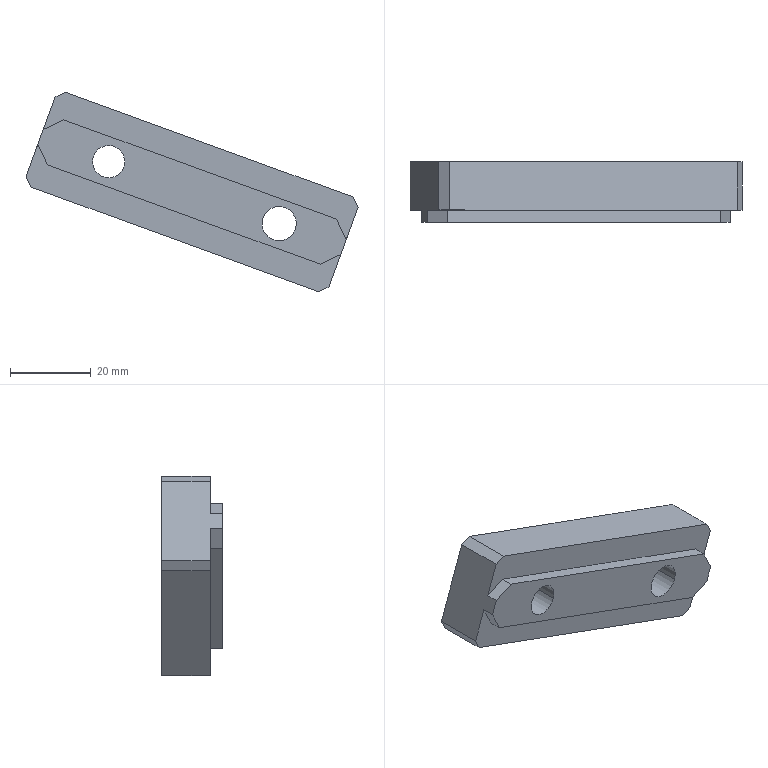Component | SolidWorks | MA060.03.03-06-8 | 1 solid | 22 faces | box 82.36 x 15 x 49.49 mm | volume 25059 mm3 | plane 18 | cylinder 4 | commonest cylinder face diameters 8.5 x2 8 x2 | material Q235A
STEP:
#1=COLOUR_RGB('',0.7922,0.8196,0.9333);
#2=FILL_AREA_STYLE_COLOUR('',#1);
#3=FILL_AREA_STYLE('',(#2));
#4=SURFACE_STYLE_FILL_AREA(#3);
#5=SURFACE_SIDE_STYLE('',(#4));
#6=SURFACE_STYLE_USAGE(.BOTH.,#5);
#7=PRESENTATION_STYLE_ASSIGNMENT((#6));
#8=CARTESIAN_POINT('',(-8.875,3.427,3.232));
#9=VERTEX_POINT('',#8);
#10=CARTESIAN_POINT('',(-8.56,3.427,3.118));
#11=VERTEX_POINT('',#10);
#12=CARTESIAN_POINT('',(-8.718,3.427,3.175));
#13=DIRECTION('',(-0.,1.,0.));
#14=DIRECTION('',(0.9397,0.,-0.342));
#15=AXIS2_PLACEMENT_3D('',#12,#13,#14);
#16=CIRCLE('',#15,0.1673);
#17=EDGE_CURVE('',#9,#11,#16,.T.);
#18=ORIENTED_EDGE('',*,*,#17,.F.);
#19=CARTESIAN_POINT('',(-8.875,4.018,3.232));
#20=VERTEX_POINT('',#19);
#21=CARTESIAN_POINT('',(-8.875,3.427,3.232));
#22=DIRECTION('',(-0.,1.,0.));
#23=VECTOR('',#22,39.37);
#24=LINE('',#21,#23);
#25=EDGE_CURVE('',#9,#20,#24,.T.);
#26=ORIENTED_EDGE('',*,*,#25,.T.);
#27=CARTESIAN_POINT('',(-8.56,4.018,3.118));
#28=VERTEX_POINT('',#27);
#29=CARTESIAN_POINT('',(-8.718,4.018,3.175));
#30=DIRECTION('',(-0.,1.,0.));
#31=DIRECTION('',(0.9397,0.,-0.342));
#32=AXIS2_PLACEMENT_3D('',#29,#30,#31);
#33=CIRCLE('',#32,0.1673);
#34=EDGE_CURVE('',#20,#28,#33,.T.);
#35=ORIENTED_EDGE('',*,*,#34,.T.);
#36=CARTESIAN_POINT('',(-8.56,3.427,3.118));
#37=DIRECTION('',(-0.,1.,0.));
#38=VECTOR('',#37,39.37);
#39=LINE('',#36,#38);
#40=EDGE_CURVE('',#11,#28,#39,.T.);
#41=ORIENTED_EDGE('',*,*,#40,.F.);
#42=EDGE_LOOP('',(#18,#26,#35,#41));
#43=FACE_OUTER_BOUND('',#42,.T.);
#44=CARTESIAN_POINT('',(-8.718,3.427,3.175));
#45=DIRECTION('',(-0.,1.,0.));
#46=DIRECTION('',(0.9397,0.,-0.342));
#47=AXIS2_PLACEMENT_3D('',#44,#45,#46);
#48=CYLINDRICAL_SURFACE('',#47,0.1673);
#49=ADVANCED_FACE('',(#43),#48,.F.);
#50=CARTESIAN_POINT('',(-10.53,3.427,3.835));
#51=VERTEX_POINT('',#50);
#52=CARTESIAN_POINT('',(-10.234,3.427,3.727));
#53=VERTEX_POINT('',#52);
#54=CARTESIAN_POINT('',(-10.382,3.427,3.781));
#55=DIRECTION('',(-0.,1.,0.));
#56=DIRECTION('',(0.9397,0.,-0.342));
#57=AXIS2_PLACEMENT_3D('',#54,#55,#56);
#58=CIRCLE('',#57,0.1575);
#59=EDGE_CURVE('',#51,#53,#58,.T.);
#60=ORIENTED_EDGE('',*,*,#59,.F.);
#61=CARTESIAN_POINT('',(-10.53,4.018,3.835));
#62=VERTEX_POINT('',#61);
#63=CARTESIAN_POINT('',(-10.53,4.018,3.835));
#64=DIRECTION('',(-0.,1.,0.));
#65=VECTOR('',#64,39.37);
#66=LINE('',#63,#65);
#67=EDGE_CURVE('',#51,#62,#66,.T.);
#68=ORIENTED_EDGE('',*,*,#67,.T.);
#69=CARTESIAN_POINT('',(-10.234,4.018,3.727));
#70=VERTEX_POINT('',#69);
#71=CARTESIAN_POINT('',(-10.382,4.018,3.781));
#72=DIRECTION('',(-0.,1.,0.));
#73=DIRECTION('',(0.9397,0.,-0.342));
#74=AXIS2_PLACEMENT_3D('',#71,#72,#73);
#75=CIRCLE('',#74,0.1575);
#76=EDGE_CURVE('',#62,#70,#75,.T.);
#77=ORIENTED_EDGE('',*,*,#76,.T.);
#78=CARTESIAN_POINT('',(-10.234,4.018,3.727));
#79=DIRECTION('',(-0.,1.,0.));
#80=VECTOR('',#79,39.37);
#81=LINE('',#78,#80);
#82=EDGE_CURVE('',#53,#70,#81,.T.);
#83=ORIENTED_EDGE('',*,*,#82,.F.);
#84=EDGE_LOOP('',(#60,#68,#77,#83));
#85=FACE_OUTER_BOUND('',#84,.T.);
#86=CARTESIAN_POINT('',(-10.382,4.018,3.781));
#87=DIRECTION('',(-0.,1.,0.));
#88=DIRECTION('',(0.9397,0.,-0.342));
#89=AXIS2_PLACEMENT_3D('',#86,#87,#88);
#90=CYLINDRICAL_SURFACE('',#89,0.1575);
#91=ADVANCED_FACE('',(#85),#90,.F.);
#92=CARTESIAN_POINT('',(-8.718,3.427,3.175));
#93=DIRECTION('',(-0.,1.,0.));
#94=DIRECTION('',(0.9397,0.,-0.342));
#95=AXIS2_PLACEMENT_3D('',#92,#93,#94);
#96=CIRCLE('',#95,0.1673);
#97=EDGE_CURVE('',#11,#9,#96,.T.);
#98=ORIENTED_EDGE('',*,*,#97,.T.);
#99=ORIENTED_EDGE('',*,*,#17,.T.);
#100=EDGE_LOOP('',(#98,#99));
#101=FACE_BOUND('',#100,.T.);
#102=CARTESIAN_POINT('',(-10.382,3.427,3.781));
#103=DIRECTION('',(-0.,1.,0.));
#104=DIRECTION('',(0.9397,0.,-0.342));
#105=AXIS2_PLACEMENT_3D('',#102,#103,#104);
#106=CIRCLE('',#105,0.1575);
#107=EDGE_CURVE('',#53,#51,#106,.T.);
#108=ORIENTED_EDGE('',*,*,#107,.T.);
#109=ORIENTED_EDGE('',*,*,#59,.T.);
#110=EDGE_LOOP('',(#108,#109));
#111=FACE_BOUND('',#110,.T.);
#112=CARTESIAN_POINT('',(-11.075,3.427,3.951));
#113=VERTEX_POINT('',#112);
#114=CARTESIAN_POINT('',(-11.022,3.427,4.095));
#115=VERTEX_POINT('',#114);
#116=CARTESIAN_POINT('',(-10.88,3.427,4.486));
#117=DIRECTION('',(0.342,0.,0.9397));
#118=VECTOR('',#117,39.37);
#119=LINE('',#116,#118);
#120=EDGE_CURVE('',#113,#115,#119,.T.);
#121=ORIENTED_EDGE('',*,*,#120,.F.);
#122=CARTESIAN_POINT('',(-10.98,3.427,3.749));
#123=VERTEX_POINT('',#122);
#124=CARTESIAN_POINT('',(-11.086,3.427,3.976));
#125=DIRECTION('',(0.4226,0.,-0.9063));
#126=VECTOR('',#125,39.37);
#127=LINE('',#124,#126);
#128=EDGE_CURVE('',#113,#123,#127,.T.);
#129=ORIENTED_EDGE('',*,*,#128,.T.);
#130=CARTESIAN_POINT('',(-8.317,3.427,2.78));
#131=VERTEX_POINT('',#130);
#132=CARTESIAN_POINT('',(-11.128,3.427,3.803));
#133=DIRECTION('',(0.9397,0.,-0.342));
#134=VECTOR('',#133,39.37);
#135=LINE('',#132,#134);
#136=EDGE_CURVE('',#123,#131,#135,.T.);
#137=ORIENTED_EDGE('',*,*,#136,.T.);
#138=CARTESIAN_POINT('',(-8.115,3.427,2.874));
#139=VERTEX_POINT('',#138);
#140=CARTESIAN_POINT('',(-8.09,3.427,2.886));
#141=DIRECTION('',(0.9063,0.,0.4226));
#142=VECTOR('',#141,39.37);
#143=LINE('',#140,#142);
#144=EDGE_CURVE('',#131,#139,#143,.T.);
#145=ORIENTED_EDGE('',*,*,#144,.T.);
#146=CARTESIAN_POINT('',(-8.062,3.427,3.018));
#147=VERTEX_POINT('',#146);
#148=CARTESIAN_POINT('',(-7.92,3.427,3.409));
#149=DIRECTION('',(-0.342,-0.,-0.9397));
#150=VECTOR('',#149,39.37);
#151=LINE('',#148,#150);
#152=EDGE_CURVE('',#147,#139,#151,.T.);
#153=ORIENTED_EDGE('',*,*,#152,.F.);
#154=CARTESIAN_POINT('',(-8.156,3.427,3.22));
#155=VERTEX_POINT('',#154);
#156=CARTESIAN_POINT('',(-8.051,3.427,2.993));
#157=DIRECTION('',(-0.4226,-0.,0.9063));
#158=VECTOR('',#157,39.37);
#159=LINE('',#156,#158);
#160=EDGE_CURVE('',#147,#155,#159,.T.);
#161=ORIENTED_EDGE('',*,*,#160,.T.);
#162=CARTESIAN_POINT('',(-10.82,3.427,4.19));
#163=VERTEX_POINT('',#162);
#164=CARTESIAN_POINT('',(-10.968,3.427,4.243));
#165=DIRECTION('',(0.9397,0.,-0.342));
#166=VECTOR('',#165,39.37);
#167=LINE('',#164,#166);
#168=EDGE_CURVE('',#163,#155,#167,.T.);
#169=ORIENTED_EDGE('',*,*,#168,.F.);
#170=CARTESIAN_POINT('',(-11.047,3.427,4.084));
#171=DIRECTION('',(-0.9063,-0.,-0.4226));
#172=VECTOR('',#171,39.37);
#173=LINE('',#170,#172);
#174=EDGE_CURVE('',#163,#115,#173,.T.);
#175=ORIENTED_EDGE('',*,*,#174,.T.);
#176=EDGE_LOOP('',(#121,#129,#137,#145,#153,#161,#169,#175));
#177=FACE_OUTER_BOUND('',#176,.T.);
#178=CARTESIAN_POINT('',(-9.568,3.427,3.485));
#179=DIRECTION('',(0.,-1.,-0.));
#180=DIRECTION('',(-0.9397,-0.,0.342));
#181=AXIS2_PLACEMENT_3D('',#178,#179,#180);
#182=PLANE('',#181);
#183=ADVANCED_FACE('',(#101,#111,#177),#182,.T.);
#184=CARTESIAN_POINT('',(-8.062,3.545,3.018));
#185=VERTEX_POINT('',#184);
#186=CARTESIAN_POINT('',(-8.062,4.018,3.018));
#187=DIRECTION('',(-0.,1.,0.));
#188=VECTOR('',#187,39.37);
#189=LINE('',#186,#188);
#190=EDGE_CURVE('',#147,#185,#189,.T.);
#191=ORIENTED_EDGE('',*,*,#190,.F.);
#192=ORIENTED_EDGE('',*,*,#152,.T.);
#193=CARTESIAN_POINT('',(-8.115,3.545,2.874));
#194=VERTEX_POINT('',#193);
#195=CARTESIAN_POINT('',(-8.115,4.018,2.874));
#196=DIRECTION('',(0.,-1.,-0.));
#197=VECTOR('',#196,39.37);
#198=LINE('',#195,#197);
#199=EDGE_CURVE('',#194,#139,#198,.T.);
#200=ORIENTED_EDGE('',*,*,#199,.F.);
#201=CARTESIAN_POINT('',(-8.23,3.545,2.558));
#202=VERTEX_POINT('',#201);
#203=CARTESIAN_POINT('',(-8.257,3.545,2.484));
#204=DIRECTION('',(0.342,-0.,0.9397));
#205=VECTOR('',#204,39.37);
#206=LINE('',#203,#205);
#207=EDGE_CURVE('',#202,#194,#206,.T.);
#208=ORIENTED_EDGE('',*,*,#207,.F.);
#209=CARTESIAN_POINT('',(-8.23,4.018,2.558));
#210=VERTEX_POINT('',#209);
#211=CARTESIAN_POINT('',(-8.23,4.018,2.558));
#212=DIRECTION('',(-0.,1.,0.));
#213=VECTOR('',#212,39.37);
#214=LINE('',#211,#213);
#215=EDGE_CURVE('',#202,#210,#214,.T.);
#216=ORIENTED_EDGE('',*,*,#215,.T.);
#217=CARTESIAN_POINT('',(-7.947,4.018,3.335));
#218=VERTEX_POINT('',#217);
#219=CARTESIAN_POINT('',(-7.92,4.018,3.409));
#220=DIRECTION('',(-0.342,-0.,-0.9397));
#221=VECTOR('',#220,39.37);
#222=LINE('',#219,#221);
#223=EDGE_CURVE('',#218,#210,#222,.T.);
#224=ORIENTED_EDGE('',*,*,#223,.F.);
#225=CARTESIAN_POINT('',(-7.947,3.545,3.335));
#226=VERTEX_POINT('',#225);
#227=CARTESIAN_POINT('',(-7.947,4.018,3.335));
#228=DIRECTION('',(0.,-1.,-0.));
#229=VECTOR('',#228,39.37);
#230=LINE('',#227,#229);
#231=EDGE_CURVE('',#218,#226,#230,.T.);
#232=ORIENTED_EDGE('',*,*,#231,.T.);
#233=CARTESIAN_POINT('',(-7.92,3.545,3.409));
#234=DIRECTION('',(0.342,0.,0.9397));
#235=VECTOR('',#234,39.37);
#236=LINE('',#233,#235);
#237=EDGE_CURVE('',#185,#226,#236,.T.);
#238=ORIENTED_EDGE('',*,*,#237,.F.);
#239=EDGE_LOOP('',(#191,#192,#200,#208,#216,#224,#232,#238));
#240=FACE_OUTER_BOUND('',#239,.T.);
#241=CARTESIAN_POINT('',(-7.92,4.018,3.409));
#242=DIRECTION('',(-0.9397,-0.,0.342));
#243=DIRECTION('',(-0.,1.,0.));
#244=AXIS2_PLACEMENT_3D('',#241,#242,#243);
#245=PLANE('',#244);
#246=ADVANCED_FACE('',(#240),#245,.F.);
#247=CARTESIAN_POINT('',(-11.075,3.545,3.951));
#248=VERTEX_POINT('',#247);
#249=CARTESIAN_POINT('',(-11.075,4.018,3.951));
#250=DIRECTION('',(-0.,1.,0.));
#251=VECTOR('',#250,39.37);
#252=LINE('',#249,#251);
#253=EDGE_CURVE('',#113,#248,#252,.T.);
#254=ORIENTED_EDGE('',*,*,#253,.F.);
#255=ORIENTED_EDGE('',*,*,#120,.T.);
#256=CARTESIAN_POINT('',(-11.022,3.545,4.095));
#257=VERTEX_POINT('',#256);
#258=CARTESIAN_POINT('',(-11.022,4.018,4.095));
#259=DIRECTION('',(0.,-1.,-0.));
#260=VECTOR('',#259,39.37);
#261=LINE('',#258,#260);
#262=EDGE_CURVE('',#257,#115,#261,.T.);
#263=ORIENTED_EDGE('',*,*,#262,.F.);
#264=CARTESIAN_POINT('',(-10.907,3.545,4.412));
#265=VERTEX_POINT('',#264);
#266=CARTESIAN_POINT('',(-10.88,3.545,4.486));
#267=DIRECTION('',(0.342,0.,0.9397));
#268=VECTOR('',#267,39.37);
#269=LINE('',#266,#268);
#270=EDGE_CURVE('',#257,#265,#269,.T.);
#271=ORIENTED_EDGE('',*,*,#270,.T.);
#272=CARTESIAN_POINT('',(-10.907,4.018,4.412));
#273=VERTEX_POINT('',#272);
#274=CARTESIAN_POINT('',(-10.907,4.018,4.412));
#275=DIRECTION('',(-0.,1.,0.));
#276=VECTOR('',#275,39.37);
#277=LINE('',#274,#276);
#278=EDGE_CURVE('',#265,#273,#277,.T.);
#279=ORIENTED_EDGE('',*,*,#278,.T.);
#280=CARTESIAN_POINT('',(-11.19,4.018,3.635));
#281=VERTEX_POINT('',#280);
#282=CARTESIAN_POINT('',(-10.88,4.018,4.486));
#283=DIRECTION('',(0.342,0.,0.9397));
#284=VECTOR('',#283,39.37);
#285=LINE('',#282,#284);
#286=EDGE_CURVE('',#281,#273,#285,.T.);
#287=ORIENTED_EDGE('',*,*,#286,.F.);
#288=CARTESIAN_POINT('',(-11.19,3.545,3.635));
#289=VERTEX_POINT('',#288);
#290=CARTESIAN_POINT('',(-11.19,4.018,3.635));
#291=DIRECTION('',(0.,-1.,-0.));
#292=VECTOR('',#291,39.37);
#293=LINE('',#290,#292);
#294=EDGE_CURVE('',#281,#289,#293,.T.);
#295=ORIENTED_EDGE('',*,*,#294,.T.);
#296=CARTESIAN_POINT('',(-11.217,3.545,3.561));
#297=DIRECTION('',(0.342,-0.,0.9397));
#298=VECTOR('',#297,39.37);
#299=LINE('',#296,#298);
#300=EDGE_CURVE('',#289,#248,#299,.T.);
#301=ORIENTED_EDGE('',*,*,#300,.T.);
#302=EDGE_LOOP('',(#254,#255,#263,#271,#279,#287,#295,#301));
#303=FACE_OUTER_BOUND('',#302,.T.);
#304=CARTESIAN_POINT('',(-10.88,4.018,4.486));
#305=DIRECTION('',(0.9397,0.,-0.342));
#306=DIRECTION('',(0.,-1.,-0.));
#307=AXIS2_PLACEMENT_3D('',#304,#305,#306);
#308=PLANE('',#307);
#309=ADVANCED_FACE('',(#303),#308,.F.);
#310=CARTESIAN_POINT('',(-10.98,3.545,3.749));
#311=VERTEX_POINT('',#310);
#312=CARTESIAN_POINT('',(-10.98,3.427,3.749));
#313=DIRECTION('',(0.,-1.,-0.));
#314=VECTOR('',#313,39.37);
#315=LINE('',#312,#314);
#316=EDGE_CURVE('',#311,#123,#315,.T.);
#317=ORIENTED_EDGE('',*,*,#316,.F.);
#318=CARTESIAN_POINT('',(-8.317,3.545,2.78));
#319=VERTEX_POINT('',#318);
#320=CARTESIAN_POINT('',(-11.128,3.545,3.803));
#321=DIRECTION('',(0.9397,0.,-0.342));
#322=VECTOR('',#321,39.37);
#323=LINE('',#320,#322);
#324=EDGE_CURVE('',#311,#319,#323,.T.);
#325=ORIENTED_EDGE('',*,*,#324,.T.);
#326=CARTESIAN_POINT('',(-8.317,3.427,2.78));
#327=DIRECTION('',(-0.,1.,0.));
#328=VECTOR('',#327,39.37);
#329=LINE('',#326,#328);
#330=EDGE_CURVE('',#131,#319,#329,.T.);
#331=ORIENTED_EDGE('',*,*,#330,.F.);
#332=ORIENTED_EDGE('',*,*,#136,.F.);
#333=EDGE_LOOP('',(#317,#325,#331,#332));
#334=FACE_OUTER_BOUND('',#333,.T.);
#335=CARTESIAN_POINT('',(-11.128,3.427,3.803));
#336=DIRECTION('',(0.342,0.,0.9397));
#337=DIRECTION('',(0.,-1.,-0.));
#338=AXIS2_PLACEMENT_3D('',#335,#336,#337);
#339=PLANE('',#338);
#340=ADVANCED_FACE('',(#334),#339,.F.);
#341=CARTESIAN_POINT('',(-8.156,3.545,3.22));
#342=VERTEX_POINT('',#341);
#343=CARTESIAN_POINT('',(-8.156,3.427,3.22));
#344=DIRECTION('',(0.,-1.,-0.));
#345=VECTOR('',#344,39.37);
#346=LINE('',#343,#345);
#347=EDGE_CURVE('',#342,#155,#346,.T.);
#348=ORIENTED_EDGE('',*,*,#347,.F.);
#349=CARTESIAN_POINT('',(-10.82,3.545,4.19));
#350=VERTEX_POINT('',#349);
#351=CARTESIAN_POINT('',(-10.968,3.545,4.243));
#352=DIRECTION('',(0.9397,0.,-0.342));
#353=VECTOR('',#352,39.37);
#354=LINE('',#351,#353);
#355=EDGE_CURVE('',#350,#342,#354,.T.);
#356=ORIENTED_EDGE('',*,*,#355,.F.);
#357=CARTESIAN_POINT('',(-10.82,3.427,4.19));
#358=DIRECTION('',(-0.,1.,0.));
#359=VECTOR('',#358,39.37);
#360=LINE('',#357,#359);
#361=EDGE_CURVE('',#163,#350,#360,.T.);
#362=ORIENTED_EDGE('',*,*,#361,.F.);
#363=ORIENTED_EDGE('',*,*,#168,.T.);
#364=EDGE_LOOP('',(#348,#356,#362,#363));
#365=FACE_OUTER_BOUND('',#364,.T.);
#366=CARTESIAN_POINT('',(-10.968,3.427,4.243));
#367=DIRECTION('',(-0.342,-0.,-0.9397));
#368=DIRECTION('',(-0.,1.,0.));
#369=AXIS2_PLACEMENT_3D('',#366,#367,#368);
#370=PLANE('',#369);
#371=ADVANCED_FACE('',(#365),#370,.F.);
#372=CARTESIAN_POINT('',(-11.143,3.545,3.534));
#373=VERTEX_POINT('',#372);
#374=CARTESIAN_POINT('',(-8.331,3.545,2.511));
#375=VERTEX_POINT('',#374);
#376=CARTESIAN_POINT('',(-11.217,3.545,3.561));
#377=DIRECTION('',(0.9397,0.,-0.342));
#378=VECTOR('',#377,39.37);
#379=LINE('',#376,#378);
#380=EDGE_CURVE('',#373,#375,#379,.T.);
#381=ORIENTED_EDGE('',*,*,#380,.F.);
#382=CARTESIAN_POINT('',(-11.143,4.018,3.534));
#383=VERTEX_POINT('',#382);
#384=CARTESIAN_POINT('',(-11.143,4.018,3.534));
#385=DIRECTION('',(-0.,1.,0.));
#386=VECTOR('',#385,39.37);
#387=LINE('',#384,#386);
#388=EDGE_CURVE('',#373,#383,#387,.T.);
#389=ORIENTED_EDGE('',*,*,#388,.T.);
#390=CARTESIAN_POINT('',(-8.331,4.018,2.511));
#391=VERTEX_POINT('',#390);
#392=CARTESIAN_POINT('',(-11.217,4.018,3.561));
#393=DIRECTION('',(-0.9397,-0.,0.342));
#394=VECTOR('',#393,39.37);
#395=LINE('',#392,#394);
#396=EDGE_CURVE('',#391,#383,#395,.T.);
#397=ORIENTED_EDGE('',*,*,#396,.F.);
#398=CARTESIAN_POINT('',(-8.331,4.018,2.511));
#399=DIRECTION('',(0.,-1.,-0.));
#400=VECTOR('',#399,39.37);
#401=LINE('',#398,#400);
#402=EDGE_CURVE('',#391,#375,#401,.T.);
#403=ORIENTED_EDGE('',*,*,#402,.T.);
#404=EDGE_LOOP('',(#381,#389,#397,#403));
#405=FACE_OUTER_BOUND('',#404,.T.);
#406=CARTESIAN_POINT('',(-11.217,4.018,3.561));
#407=DIRECTION('',(0.342,0.,0.9397));
#408=DIRECTION('',(0.,-1.,-0.));
#409=AXIS2_PLACEMENT_3D('',#406,#407,#408);
#410=PLANE('',#409);
#411=ADVANCED_FACE('',(#405),#410,.F.);
#412=CARTESIAN_POINT('',(-10.806,4.018,4.459));
#413=VERTEX_POINT('',#412);
#414=CARTESIAN_POINT('',(-7.994,4.018,3.435));
#415=VERTEX_POINT('',#414);
#416=CARTESIAN_POINT('',(-10.88,4.018,4.486));
#417=DIRECTION('',(0.9397,0.,-0.342));
#418=VECTOR('',#417,39.37);
#419=LINE('',#416,#418);
#420=EDGE_CURVE('',#413,#415,#419,.T.);
#421=ORIENTED_EDGE('',*,*,#420,.F.);
#422=CARTESIAN_POINT('',(-10.806,3.545,4.459));
#423=VERTEX_POINT('',#422);
#424=CARTESIAN_POINT('',(-10.806,4.018,4.459));
#425=DIRECTION('',(0.,-1.,-0.));
#426=VECTOR('',#425,39.37);
#427=LINE('',#424,#426);
#428=EDGE_CURVE('',#413,#423,#427,.T.);
#429=ORIENTED_EDGE('',*,*,#428,.T.);
#430=CARTESIAN_POINT('',(-7.994,3.545,3.435));
#431=VERTEX_POINT('',#430);
#432=CARTESIAN_POINT('',(-10.88,3.545,4.486));
#433=DIRECTION('',(0.9397,0.,-0.342));
#434=VECTOR('',#433,39.37);
#435=LINE('',#432,#434);
#436=EDGE_CURVE('',#423,#431,#435,.T.);
#437=ORIENTED_EDGE('',*,*,#436,.T.);
#438=CARTESIAN_POINT('',(-7.994,4.018,3.435));
#439=DIRECTION('',(-0.,1.,0.));
#440=VECTOR('',#439,39.37);
#441=LINE('',#438,#440);
#442=EDGE_CURVE('',#431,#415,#441,.T.);
#443=ORIENTED_EDGE('',*,*,#442,.T.);
#444=EDGE_LOOP('',(#421,#429,#437,#443));
#445=FACE_OUTER_BOUND('',#444,.T.);
#446=CARTESIAN_POINT('',(-10.88,4.018,4.486));
#447=DIRECTION('',(-0.342,-0.,-0.9397));
#448=DIRECTION('',(-0.,1.,0.));
#449=AXIS2_PLACEMENT_3D('',#446,#447,#448);
#450=PLANE('',#449);
#451=ADVANCED_FACE('',(#445),#450,.F.);
#452=CARTESIAN_POINT('',(-8.718,4.018,3.175));
#453=DIRECTION('',(-0.,1.,0.));
#454=DIRECTION('',(0.9397,0.,-0.342));
#455=AXIS2_PLACEMENT_3D('',#452,#453,#454);
#456=CIRCLE('',#455,0.1673);
#457=EDGE_CURVE('',#28,#20,#456,.T.);
#458=ORIENTED_EDGE('',*,*,#457,.F.);
#459=ORIENTED_EDGE('',*,*,#34,.F.);
#460=EDGE_LOOP('',(#458,#459));
#461=FACE_BOUND('',#460,.T.);
#462=CARTESIAN_POINT('',(-10.382,4.018,3.781));
#463=DIRECTION('',(-0.,1.,0.));
#464=DIRECTION('',(0.9397,0.,-0.342));
#465=AXIS2_PLACEMENT_3D('',#462,#463,#464);
#466=CIRCLE('',#465,0.1575);
#467=EDGE_CURVE('',#70,#62,#466,.T.);
#468=ORIENTED_EDGE('',*,*,#467,.F.);
#469=ORIENTED_EDGE('',*,*,#76,.F.);
#470=EDGE_LOOP('',(#468,#469));
#471=FACE_BOUND('',#470,.T.);
#472=ORIENTED_EDGE('',*,*,#286,.T.);
#473=CARTESIAN_POINT('',(-10.806,4.018,4.459));
#474=DIRECTION('',(0.9063,0.,0.4226));
#475=VECTOR('',#474,39.37);
#476=LINE('',#473,#475);
#477=EDGE_CURVE('',#273,#413,#476,.T.);
#478=ORIENTED_EDGE('',*,*,#477,.T.);
#479=ORIENTED_EDGE('',*,*,#420,.T.);
#480=CARTESIAN_POINT('',(-7.947,4.018,3.335));
#481=DIRECTION('',(0.4226,0.,-0.9063));
#482=VECTOR('',#481,39.37);
#483=LINE('',#480,#482);
#484=EDGE_CURVE('',#415,#218,#483,.T.);
#485=ORIENTED_EDGE('',*,*,#484,.T.);
#486=ORIENTED_EDGE('',*,*,#223,.T.);
#487=CARTESIAN_POINT('',(-8.331,4.018,2.511));
#488=DIRECTION('',(-0.9063,-0.,-0.4226));
#489=VECTOR('',#488,39.37);
#490=LINE('',#487,#489);
#491=EDGE_CURVE('',#210,#391,#490,.T.);
#492=ORIENTED_EDGE('',*,*,#491,.T.);
#493=ORIENTED_EDGE('',*,*,#396,.T.);
#494=CARTESIAN_POINT('',(-11.19,4.018,3.635));
#495=DIRECTION('',(-0.4226,-0.,0.9063));
#496=VECTOR('',#495,39.37);
#497=LINE('',#494,#496);
#498=EDGE_CURVE('',#383,#281,#497,.T.);
#499=ORIENTED_EDGE('',*,*,#498,.T.);
#500=EDGE_LOOP('',(#472,#478,#479,#485,#486,#492,#493,#499));
#501=FACE_OUTER_BOUND('',#500,.T.);
#502=CARTESIAN_POINT('',(-9.568,4.018,3.485));
#503=DIRECTION('',(0.,-1.,-0.));
#504=DIRECTION('',(-0.9397,-0.,0.342));
#505=AXIS2_PLACEMENT_3D('',#502,#503,#504);
#506=PLANE('',#505);
#507=ADVANCED_FACE('',(#461,#471,#501),#506,.F.);
#508=ORIENTED_EDGE('',*,*,#67,.F.);
#509=ORIENTED_EDGE('',*,*,#107,.F.);
#510=ORIENTED_EDGE('',*,*,#82,.T.);
#511=ORIENTED_EDGE('',*,*,#467,.T.);
#512=EDGE_LOOP('',(#508,#509,#510,#511));
#513=FACE_OUTER_BOUND('',#512,.T.);
#514=CARTESIAN_POINT('',(-10.382,4.018,3.781));
#515=DIRECTION('',(-0.,1.,0.));
#516=DIRECTION('',(0.9397,0.,-0.342));
#517=AXIS2_PLACEMENT_3D('',#514,#515,#516);
#518=CYLINDRICAL_SURFACE('',#517,0.1575);
#519=ADVANCED_FACE('',(#513),#518,.F.);
#520=ORIENTED_EDGE('',*,*,#324,.F.);
#521=CARTESIAN_POINT('',(-11.086,3.545,3.976));
#522=DIRECTION('',(0.4226,0.,-0.9063));
#523=VECTOR('',#522,39.37);
#524=LINE('',#521,#523);
#525=EDGE_CURVE('',#248,#311,#524,.T.);
#526=ORIENTED_EDGE('',*,*,#525,.F.);
#527=ORIENTED_EDGE('',*,*,#300,.F.);
#528=CARTESIAN_POINT('',(-11.19,3.545,3.635));
#529=DIRECTION('',(0.4226,0.,-0.9063));
#530=VECTOR('',#529,39.37);
#531=LINE('',#528,#530);
#532=EDGE_CURVE('',#289,#373,#531,.T.);
#533=ORIENTED_EDGE('',*,*,#532,.T.);
#534=ORIENTED_EDGE('',*,*,#380,.T.);
#535=CARTESIAN_POINT('',(-8.331,3.545,2.511));
#536=DIRECTION('',(0.9063,-0.,0.4226));
#537=VECTOR('',#536,39.37);
#538=LINE('',#535,#537);
#539=EDGE_CURVE('',#375,#202,#538,.T.);
#540=ORIENTED_EDGE('',*,*,#539,.T.);
#541=ORIENTED_EDGE('',*,*,#207,.T.);
#542=CARTESIAN_POINT('',(-8.09,3.545,2.886));
#543=DIRECTION('',(0.9063,0.,0.4226));
#544=VECTOR('',#543,39.37);
#545=LINE('',#542,#544);
#546=EDGE_CURVE('',#319,#194,#545,.T.);
#547=ORIENTED_EDGE('',*,*,#546,.F.);
#548=EDGE_LOOP('',(#520,#526,#527,#533,#534,#540,#541,#547));
#549=FACE_OUTER_BOUND('',#548,.T.);
#550=CARTESIAN_POINT('',(-11.217,3.545,3.561));
#551=DIRECTION('',(-0.,1.,0.));
#552=DIRECTION('',(0.342,-0.,0.9397));
#553=AXIS2_PLACEMENT_3D('',#550,#551,#552);
#554=PLANE('',#553);
#555=ADVANCED_FACE('',(#549),#554,.F.);
#556=CARTESIAN_POINT('',(-11.047,3.545,4.084));
#557=DIRECTION('',(-0.9063,-0.,-0.4226));
#558=VECTOR('',#557,39.37);
#559=LINE('',#556,#558);
#560=EDGE_CURVE('',#350,#257,#559,.T.);
#561=ORIENTED_EDGE('',*,*,#560,.F.);
#562=ORIENTED_EDGE('',*,*,#355,.T.);
#563=CARTESIAN_POINT('',(-8.051,3.545,2.993));
#564=DIRECTION('',(-0.4226,-0.,0.9063));
#565=VECTOR('',#564,39.37);
#566=LINE('',#563,#565);
#567=EDGE_CURVE('',#185,#342,#566,.T.);
#568=ORIENTED_EDGE('',*,*,#567,.F.);
#569=ORIENTED_EDGE('',*,*,#237,.T.);
#570=CARTESIAN_POINT('',(-7.947,3.545,3.335));
#571=DIRECTION('',(-0.4226,0.,0.9063));
#572=VECTOR('',#571,39.37);
#573=LINE('',#570,#572);
#574=EDGE_CURVE('',#226,#431,#573,.T.);
#575=ORIENTED_EDGE('',*,*,#574,.T.);
#576=ORIENTED_EDGE('',*,*,#436,.F.);
#577=CARTESIAN_POINT('',(-10.806,3.545,4.459));
#578=DIRECTION('',(-0.9063,-0.,-0.4226));
#579=VECTOR('',#578,39.37);
#580=LINE('',#577,#579);
#581=EDGE_CURVE('',#423,#265,#580,.T.);
#582=ORIENTED_EDGE('',*,*,#581,.T.);
#583=ORIENTED_EDGE('',*,*,#270,.F.);
#584=EDGE_LOOP('',(#561,#562,#568,#569,#575,#576,#582,#583));
#585=FACE_OUTER_BOUND('',#584,.T.);
#586=CARTESIAN_POINT('',(-10.88,3.545,4.486));
#587=DIRECTION('',(-0.,1.,-0.));
#588=DIRECTION('',(0.342,0.,0.9397));
#589=AXIS2_PLACEMENT_3D('',#586,#587,#588);
#590=PLANE('',#589);
#591=ADVANCED_FACE('',(#585),#590,.F.);
#592=ORIENTED_EDGE('',*,*,#25,.F.);
#593=ORIENTED_EDGE('',*,*,#97,.F.);
#594=ORIENTED_EDGE('',*,*,#40,.T.);
#595=ORIENTED_EDGE('',*,*,#457,.T.);
#596=EDGE_LOOP('',(#592,#593,#594,#595));
#597=FACE_OUTER_BOUND('',#596,.T.);
#598=CARTESIAN_POINT('',(-8.718,3.427,3.175));
#599=DIRECTION('',(-0.,1.,0.));
#600=DIRECTION('',(0.9397,0.,-0.342));
#601=AXIS2_PLACEMENT_3D('',#598,#599,#600);
#602=CYLINDRICAL_SURFACE('',#601,0.1673);
#603=ADVANCED_FACE('',(#597),#602,.F.);
#604=ORIENTED_EDGE('',*,*,#477,.F.);
#605=ORIENTED_EDGE('',*,*,#278,.F.);
#606=ORIENTED_EDGE('',*,*,#581,.F.);
#607=ORIENTED_EDGE('',*,*,#428,.F.);
#608=EDGE_LOOP('',(#604,#605,#606,#607));
#609=FACE_OUTER_BOUND('',#608,.T.);
#610=CARTESIAN_POINT('',(-10.806,4.018,4.459));
#611=DIRECTION('',(0.4226,0.,-0.9063));
#612=DIRECTION('',(0.,-1.,-0.));
#613=AXIS2_PLACEMENT_3D('',#610,#611,#612);
#614=PLANE('',#613);
#615=ADVANCED_FACE('',(#609),#614,.F.);
#616=ORIENTED_EDGE('',*,*,#498,.F.);
#617=ORIENTED_EDGE('',*,*,#388,.F.);
#618=ORIENTED_EDGE('',*,*,#532,.F.);
#619=ORIENTED_EDGE('',*,*,#294,.F.);
#620=EDGE_LOOP('',(#616,#617,#618,#619));
#621=FACE_OUTER_BOUND('',#620,.T.);
#622=CARTESIAN_POINT('',(-11.19,4.018,3.635));
#623=DIRECTION('',(0.9063,0.,0.4226));
#624=DIRECTION('',(0.,-1.,-0.));
#625=AXIS2_PLACEMENT_3D('',#622,#623,#624);
#626=PLANE('',#625);
#627=ADVANCED_FACE('',(#621),#626,.F.);
#628=ORIENTED_EDGE('',*,*,#491,.F.);
#629=ORIENTED_EDGE('',*,*,#215,.F.);
#630=ORIENTED_EDGE('',*,*,#539,.F.);
#631=ORIENTED_EDGE('',*,*,#402,.F.);
#632=EDGE_LOOP('',(#628,#629,#630,#631));
#633=FACE_OUTER_BOUND('',#632,.T.);
#634=CARTESIAN_POINT('',(-8.331,4.018,2.511));
#635=DIRECTION('',(-0.4226,-0.,0.9063));
#636=DIRECTION('',(0.,-1.,-0.));
#637=AXIS2_PLACEMENT_3D('',#634,#635,#636);
#638=PLANE('',#637);
#639=ADVANCED_FACE('',(#633),#638,.F.);
#640=ORIENTED_EDGE('',*,*,#484,.F.);
#641=ORIENTED_EDGE('',*,*,#442,.F.);
#642=ORIENTED_EDGE('',*,*,#574,.F.);
#643=ORIENTED_EDGE('',*,*,#231,.F.);
#644=EDGE_LOOP('',(#640,#641,#642,#643));
#645=FACE_OUTER_BOUND('',#644,.T.);
#646=CARTESIAN_POINT('',(-7.947,4.018,3.335));
#647=DIRECTION('',(-0.9063,-0.,-0.4226));
#648=DIRECTION('',(0.,-1.,-0.));
#649=AXIS2_PLACEMENT_3D('',#646,#647,#648);
#650=PLANE('',#649);
#651=ADVANCED_FACE('',(#645),#650,.F.);
#652=ORIENTED_EDGE('',*,*,#262,.T.);
#653=ORIENTED_EDGE('',*,*,#174,.F.);
#654=ORIENTED_EDGE('',*,*,#361,.T.);
#655=ORIENTED_EDGE('',*,*,#560,.T.);
#656=EDGE_LOOP('',(#652,#653,#654,#655));
#657=FACE_OUTER_BOUND('',#656,.T.);
#658=CARTESIAN_POINT('',(-11.047,3.545,4.084));
#659=DIRECTION('',(-0.4226,-0.,0.9063));
#660=DIRECTION('',(0.9063,0.,0.4226));
#661=AXIS2_PLACEMENT_3D('',#658,#659,#660);
#662=PLANE('',#661);
#663=ADVANCED_FACE('',(#657),#662,.T.);
#664=ORIENTED_EDGE('',*,*,#253,.T.);
#665=ORIENTED_EDGE('',*,*,#525,.T.);
#666=ORIENTED_EDGE('',*,*,#316,.T.);
#667=ORIENTED_EDGE('',*,*,#128,.F.);
#668=EDGE_LOOP('',(#664,#665,#666,#667));
#669=FACE_OUTER_BOUND('',#668,.T.);
#670=CARTESIAN_POINT('',(-11.086,3.545,3.976));
#671=DIRECTION('',(-0.9063,-0.,-0.4226));
#672=DIRECTION('',(-0.4226,-0.,0.9063));
#673=AXIS2_PLACEMENT_3D('',#670,#671,#672);
#674=PLANE('',#673);
#675=ADVANCED_FACE('',(#669),#674,.T.);
#676=ORIENTED_EDGE('',*,*,#199,.T.);
#677=ORIENTED_EDGE('',*,*,#144,.F.);
#678=ORIENTED_EDGE('',*,*,#330,.T.);
#679=ORIENTED_EDGE('',*,*,#546,.T.);
#680=EDGE_LOOP('',(#676,#677,#678,#679));
#681=FACE_OUTER_BOUND('',#680,.T.);
#682=CARTESIAN_POINT('',(-8.09,3.545,2.886));
#683=DIRECTION('',(0.4226,0.,-0.9063));
#684=DIRECTION('',(-0.9063,-0.,-0.4226));
#685=AXIS2_PLACEMENT_3D('',#682,#683,#684);
#686=PLANE('',#685);
#687=ADVANCED_FACE('',(#681),#686,.T.);
#688=ORIENTED_EDGE('',*,*,#190,.T.);
#689=ORIENTED_EDGE('',*,*,#567,.T.);
#690=ORIENTED_EDGE('',*,*,#347,.T.);
#691=ORIENTED_EDGE('',*,*,#160,.F.);
#692=EDGE_LOOP('',(#688,#689,#690,#691));
#693=FACE_OUTER_BOUND('',#692,.T.);
#694=CARTESIAN_POINT('',(-8.051,3.545,2.993));
#695=DIRECTION('',(0.9063,0.,0.4226));
#696=DIRECTION('',(0.4226,0.,-0.9063));
#697=AXIS2_PLACEMENT_3D('',#694,#695,#696);
#698=PLANE('',#697);
#699=ADVANCED_FACE('',(#693),#698,.T.);
#700=CLOSED_SHELL('',(#49,#91,#183,#246,#309,#340,#371,#411,#451,#507,#519,#555,#591,#603,#615,#627,#639,#651,#663,#675,#687,#699));
#701=MANIFOLD_SOLID_BREP('',#700);
#702=STYLED_ITEM('',(#7),#701);
#703=PRESENTATION_LAYER_ASSIGNMENT('','',(#702));
#704=CARTESIAN_POINT('',(0.,0.,0.));
#705=DIRECTION('',(0.,0.,1.));
#706=DIRECTION('',(1.,0.,0.));
#707=AXIS2_PLACEMENT_3D('',#704,#705,#706);
#708=(LENGTH_UNIT()NAMED_UNIT(*)SI_UNIT($,.METRE.));
#709=LENGTH_MEASURE_WITH_UNIT(LENGTH_MEASURE(0.0254),#708);
#710=DIMENSIONAL_EXPONENTS(1.,0.,0.,0.,0.,0.,0.);
#711=(CONVERSION_BASED_UNIT('',#709)LENGTH_UNIT()NAMED_UNIT(#710));
#712=UNCERTAINTY_MEASURE_WITH_UNIT(LENGTH_MEASURE(0.00001),#711,'','');
#713=(NAMED_UNIT(*)PLANE_ANGLE_UNIT()SI_UNIT($,.RADIAN.));
#714=(NAMED_UNIT(*)SI_UNIT($,.STERADIAN.)SOLID_ANGLE_UNIT());
#715=(GEOMETRIC_REPRESENTATION_CONTEXT(3)GLOBAL_UNCERTAINTY_ASSIGNED_CONTEXT((#712))GLOBAL_UNIT_ASSIGNED_CONTEXT((#711,#713,#714))REPRESENTATION_CONTEXT('',''));
#716=ADVANCED_BREP_SHAPE_REPRESENTATION('',(#701,#707),#715);
#717=(LENGTH_UNIT()NAMED_UNIT(*)SI_UNIT($,.METRE.));
#718=LENGTH_MEASURE_WITH_UNIT(LENGTH_MEASURE(0.0254),#717);
#719=DIMENSIONAL_EXPONENTS(1.,0.,0.,0.,0.,0.,0.);
#720=(CONVERSION_BASED_UNIT('',#718)LENGTH_UNIT()NAMED_UNIT(#719));
#721=UNCERTAINTY_MEASURE_WITH_UNIT(LENGTH_MEASURE(0.00001),#720,'','');
#722=(NAMED_UNIT(*)PLANE_ANGLE_UNIT()SI_UNIT($,.RADIAN.));
#723=(NAMED_UNIT(*)SI_UNIT($,.STERADIAN.)SOLID_ANGLE_UNIT());
#724=(GEOMETRIC_REPRESENTATION_CONTEXT(3)GLOBAL_UNCERTAINTY_ASSIGNED_CONTEXT((#721))GLOBAL_UNIT_ASSIGNED_CONTEXT((#720,#722,#723))REPRESENTATION_CONTEXT('',''));
#725=MECHANICAL_DESIGN_GEOMETRIC_PRESENTATION_REPRESENTATION('',(#702),#724);